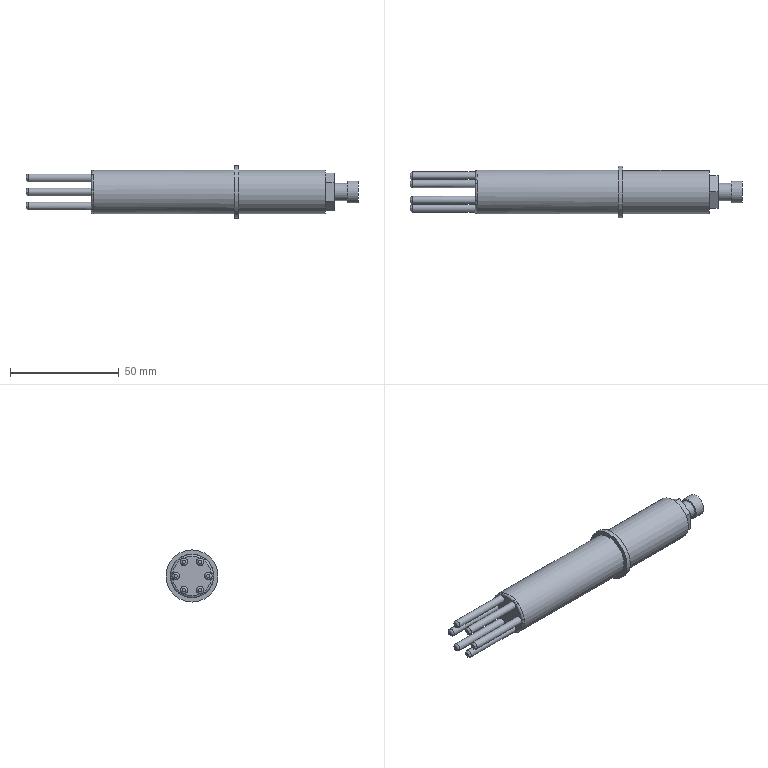Component | NX | SHAFT_01 | 1 solid | 48 faces | volume 37385 mm3 | plane 19 | spline 12 | cylinder 11 | torus 6 | commonest cylinder face diameters 3.5 x6 20 x2 24 x1 8 x1 10 x1